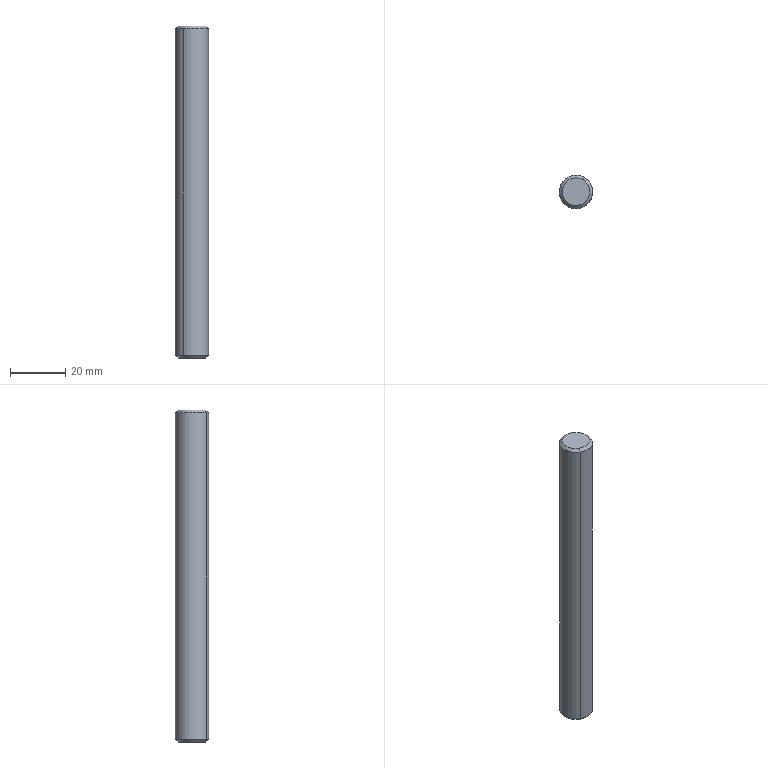Component | SolidWorks | DoubleFilmTransport-1_AdjustmentRod-1 | 1 solid | 8 faces | box 12 x 12 x 120 mm | volume 13536 mm3 | cone 4 | cylinder 2 | plane 2 | commonest cylinder face diameters 12 x2
build123d program:
from build123d import *


with BuildPart() as part:
    # Sketch1 → Revolve1 (revolve)
    with BuildSketch(Plane(origin=(0, 0, 0), x_dir=(1, 0, 0), z_dir=(0, 1, 0))):
        Polygon((5, 60), (0, 60), (0, -60), (5, -60), (6, -59), (6, 59), align=None)
    revolve(axis=Axis((0, 0, -60), (0, 0, 1)))


solid = part.part

# Placed as in the assembly
solid = solid.moved(Location((-298.746, 95.373, -1.5), (0, 0, 0)))
STEP:
#1=COLOUR_RGB('',0.7922,0.8196,0.9333);
#2=FILL_AREA_STYLE_COLOUR('',#1);
#3=FILL_AREA_STYLE('',(#2));
#4=SURFACE_STYLE_FILL_AREA(#3);
#5=SURFACE_SIDE_STYLE('',(#4));
#6=SURFACE_STYLE_USAGE(.BOTH.,#5);
#7=PRESENTATION_STYLE_ASSIGNMENT((#6));
#8=CARTESIAN_POINT('',(-11.863,3.586,2.303));
#9=VERTEX_POINT('',#8);
#10=CARTESIAN_POINT('',(-11.661,3.924,2.303));
#11=VERTEX_POINT('',#10);
#12=CARTESIAN_POINT('',(-11.762,3.755,2.303));
#13=DIRECTION('',(0.,0.,1.));
#14=DIRECTION('',(-0.5123,-0.8588,0.));
#15=AXIS2_PLACEMENT_3D('',#12,#13,#14);
#16=CIRCLE('',#15,0.1969);
#17=EDGE_CURVE('',#9,#11,#16,.T.);
#18=ORIENTED_EDGE('',*,*,#17,.F.);
#19=CARTESIAN_POINT('',(-11.883,3.552,2.264));
#20=VERTEX_POINT('',#19);
#21=CARTESIAN_POINT('',(-11.863,3.586,2.303));
#22=DIRECTION('',(-0.3623,-0.6073,-0.7071));
#23=VECTOR('',#22,39.37);
#24=LINE('',#21,#23);
#25=EDGE_CURVE('',#9,#20,#24,.T.);
#26=ORIENTED_EDGE('',*,*,#25,.T.);
#27=CARTESIAN_POINT('',(-11.641,3.958,2.264));
#28=VERTEX_POINT('',#27);
#29=CARTESIAN_POINT('',(-11.762,3.755,2.264));
#30=DIRECTION('',(0.,0.,1.));
#31=DIRECTION('',(-0.5123,-0.8588,0.));
#32=AXIS2_PLACEMENT_3D('',#29,#30,#31);
#33=CIRCLE('',#32,0.2362);
#34=EDGE_CURVE('',#20,#28,#33,.T.);
#35=ORIENTED_EDGE('',*,*,#34,.T.);
#36=CARTESIAN_POINT('',(-11.661,3.924,2.303));
#37=DIRECTION('',(0.3623,0.6073,-0.7071));
#38=VECTOR('',#37,39.37);
#39=LINE('',#36,#38);
#40=EDGE_CURVE('',#11,#28,#39,.T.);
#41=ORIENTED_EDGE('',*,*,#40,.F.);
#42=EDGE_LOOP('',(#18,#26,#35,#41));
#43=FACE_OUTER_BOUND('',#42,.T.);
#44=CARTESIAN_POINT('',(-11.762,3.755,2.303));
#45=DIRECTION('',(0.,0.,-1.));
#46=DIRECTION('',(0.5123,0.8588,0.));
#47=AXIS2_PLACEMENT_3D('',#44,#45,#46);
#48=CONICAL_SURFACE('',#47,0.1969,0.7854);
#49=ADVANCED_FACE('',(#43),#48,.T.);
#50=CARTESIAN_POINT('',(-11.883,3.552,-2.382));
#51=VERTEX_POINT('',#50);
#52=CARTESIAN_POINT('',(-11.641,3.958,-2.382));
#53=VERTEX_POINT('',#52);
#54=CARTESIAN_POINT('',(-11.762,3.755,-2.382));
#55=DIRECTION('',(0.,0.,1.));
#56=DIRECTION('',(-0.5123,-0.8588,0.));
#57=AXIS2_PLACEMENT_3D('',#54,#55,#56);
#58=CIRCLE('',#57,0.2362);
#59=EDGE_CURVE('',#51,#53,#58,.T.);
#60=ORIENTED_EDGE('',*,*,#59,.T.);
#61=CARTESIAN_POINT('',(-11.641,3.958,-2.421));
#62=DIRECTION('',(0.,0.,1.));
#63=VECTOR('',#62,39.37);
#64=LINE('',#61,#63);
#65=EDGE_CURVE('',#53,#28,#64,.T.);
#66=ORIENTED_EDGE('',*,*,#65,.T.);
#67=ORIENTED_EDGE('',*,*,#34,.F.);
#68=CARTESIAN_POINT('',(-11.883,3.552,-2.421));
#69=DIRECTION('',(0.,0.,1.));
#70=VECTOR('',#69,39.37);
#71=LINE('',#68,#70);
#72=EDGE_CURVE('',#51,#20,#71,.T.);
#73=ORIENTED_EDGE('',*,*,#72,.F.);
#74=EDGE_LOOP('',(#60,#66,#67,#73));
#75=FACE_OUTER_BOUND('',#74,.T.);
#76=CARTESIAN_POINT('',(-11.762,3.755,-2.421));
#77=DIRECTION('',(0.,0.,1.));
#78=DIRECTION('',(-0.5123,-0.8588,0.));
#79=AXIS2_PLACEMENT_3D('',#76,#77,#78);
#80=CYLINDRICAL_SURFACE('',#79,0.2362);
#81=ADVANCED_FACE('',(#75),#80,.T.);
#82=CARTESIAN_POINT('',(-11.863,3.586,-2.421));
#83=VERTEX_POINT('',#82);
#84=CARTESIAN_POINT('',(-11.661,3.924,-2.421));
#85=VERTEX_POINT('',#84);
#86=CARTESIAN_POINT('',(-11.762,3.755,-2.421));
#87=DIRECTION('',(0.,0.,1.));
#88=DIRECTION('',(-0.5123,-0.8588,0.));
#89=AXIS2_PLACEMENT_3D('',#86,#87,#88);
#90=CIRCLE('',#89,0.1969);
#91=EDGE_CURVE('',#83,#85,#90,.T.);
#92=ORIENTED_EDGE('',*,*,#91,.T.);
#93=CARTESIAN_POINT('',(-11.641,3.958,-2.382));
#94=DIRECTION('',(0.3623,0.6073,0.7071));
#95=VECTOR('',#94,39.37);
#96=LINE('',#93,#95);
#97=EDGE_CURVE('',#85,#53,#96,.T.);
#98=ORIENTED_EDGE('',*,*,#97,.T.);
#99=ORIENTED_EDGE('',*,*,#59,.F.);
#100=CARTESIAN_POINT('',(-11.883,3.552,-2.382));
#101=DIRECTION('',(-0.3623,-0.6073,0.7071));
#102=VECTOR('',#101,39.37);
#103=LINE('',#100,#102);
#104=EDGE_CURVE('',#83,#51,#103,.T.);
#105=ORIENTED_EDGE('',*,*,#104,.F.);
#106=EDGE_LOOP('',(#92,#98,#99,#105));
#107=FACE_OUTER_BOUND('',#106,.T.);
#108=CARTESIAN_POINT('',(-11.762,3.755,-2.382));
#109=DIRECTION('',(0.,0.,1.));
#110=DIRECTION('',(-0.5123,-0.8588,0.));
#111=AXIS2_PLACEMENT_3D('',#108,#109,#110);
#112=CONICAL_SURFACE('',#111,0.2362,0.7854);
#113=ADVANCED_FACE('',(#107),#112,.T.);
#114=ORIENTED_EDGE('',*,*,#97,.F.);
#115=CARTESIAN_POINT('',(-11.762,3.755,-2.421));
#116=DIRECTION('',(0.,0.,1.));
#117=DIRECTION('',(-0.5123,-0.8588,0.));
#118=AXIS2_PLACEMENT_3D('',#115,#116,#117);
#119=CIRCLE('',#118,0.1969);
#120=EDGE_CURVE('',#85,#83,#119,.T.);
#121=ORIENTED_EDGE('',*,*,#120,.T.);
#122=ORIENTED_EDGE('',*,*,#104,.T.);
#123=CARTESIAN_POINT('',(-11.762,3.755,-2.382));
#124=DIRECTION('',(0.,0.,1.));
#125=DIRECTION('',(-0.5123,-0.8588,0.));
#126=AXIS2_PLACEMENT_3D('',#123,#124,#125);
#127=CIRCLE('',#126,0.2362);
#128=EDGE_CURVE('',#53,#51,#127,.T.);
#129=ORIENTED_EDGE('',*,*,#128,.F.);
#130=EDGE_LOOP('',(#114,#121,#122,#129));
#131=FACE_OUTER_BOUND('',#130,.T.);
#132=CARTESIAN_POINT('',(-11.762,3.755,-2.382));
#133=DIRECTION('',(0.,0.,1.));
#134=DIRECTION('',(-0.5123,-0.8588,0.));
#135=AXIS2_PLACEMENT_3D('',#132,#133,#134);
#136=CONICAL_SURFACE('',#135,0.2362,0.7854);
#137=ADVANCED_FACE('',(#131),#136,.T.);
#138=ORIENTED_EDGE('',*,*,#65,.F.);
#139=ORIENTED_EDGE('',*,*,#128,.T.);
#140=ORIENTED_EDGE('',*,*,#72,.T.);
#141=CARTESIAN_POINT('',(-11.762,3.755,2.264));
#142=DIRECTION('',(0.,0.,1.));
#143=DIRECTION('',(-0.5123,-0.8588,0.));
#144=AXIS2_PLACEMENT_3D('',#141,#142,#143);
#145=CIRCLE('',#144,0.2362);
#146=EDGE_CURVE('',#28,#20,#145,.T.);
#147=ORIENTED_EDGE('',*,*,#146,.F.);
#148=EDGE_LOOP('',(#138,#139,#140,#147));
#149=FACE_OUTER_BOUND('',#148,.T.);
#150=CARTESIAN_POINT('',(-11.762,3.755,-2.421));
#151=DIRECTION('',(0.,0.,1.));
#152=DIRECTION('',(-0.5123,-0.8588,0.));
#153=AXIS2_PLACEMENT_3D('',#150,#151,#152);
#154=CYLINDRICAL_SURFACE('',#153,0.2362);
#155=ADVANCED_FACE('',(#149),#154,.T.);
#156=ORIENTED_EDGE('',*,*,#25,.F.);
#157=CARTESIAN_POINT('',(-11.762,3.755,2.303));
#158=DIRECTION('',(0.,0.,1.));
#159=DIRECTION('',(-0.5123,-0.8588,0.));
#160=AXIS2_PLACEMENT_3D('',#157,#158,#159);
#161=CIRCLE('',#160,0.1969);
#162=EDGE_CURVE('',#11,#9,#161,.T.);
#163=ORIENTED_EDGE('',*,*,#162,.F.);
#164=ORIENTED_EDGE('',*,*,#40,.T.);
#165=ORIENTED_EDGE('',*,*,#146,.T.);
#166=EDGE_LOOP('',(#156,#163,#164,#165));
#167=FACE_OUTER_BOUND('',#166,.T.);
#168=CARTESIAN_POINT('',(-11.762,3.755,2.303));
#169=DIRECTION('',(0.,0.,-1.));
#170=DIRECTION('',(0.5123,0.8588,0.));
#171=AXIS2_PLACEMENT_3D('',#168,#169,#170);
#172=CONICAL_SURFACE('',#171,0.1969,0.7854);
#173=ADVANCED_FACE('',(#167),#172,.T.);
#174=ORIENTED_EDGE('',*,*,#162,.T.);
#175=ORIENTED_EDGE('',*,*,#17,.T.);
#176=EDGE_LOOP('',(#174,#175));
#177=FACE_OUTER_BOUND('',#176,.T.);
#178=CARTESIAN_POINT('',(-11.762,3.755,2.303));
#179=DIRECTION('',(0.,0.,1.));
#180=DIRECTION('',(-0.5123,-0.8588,0.));
#181=AXIS2_PLACEMENT_3D('',#178,#179,#180);
#182=PLANE('',#181);
#183=ADVANCED_FACE('',(#177),#182,.T.);
#184=ORIENTED_EDGE('',*,*,#91,.F.);
#185=ORIENTED_EDGE('',*,*,#120,.F.);
#186=EDGE_LOOP('',(#184,#185));
#187=FACE_OUTER_BOUND('',#186,.T.);
#188=CARTESIAN_POINT('',(-11.863,3.586,-2.421));
#189=DIRECTION('',(0.,0.,-1.));
#190=DIRECTION('',(0.5123,0.8588,0.));
#191=AXIS2_PLACEMENT_3D('',#188,#189,#190);
#192=PLANE('',#191);
#193=ADVANCED_FACE('',(#187),#192,.T.);
#194=CLOSED_SHELL('',(#49,#81,#113,#137,#155,#173,#183,#193));
#195=MANIFOLD_SOLID_BREP('',#194);
#196=STYLED_ITEM('',(#7),#195);
#197=(LENGTH_UNIT()NAMED_UNIT(*)SI_UNIT($,.METRE.));
#198=LENGTH_MEASURE_WITH_UNIT(LENGTH_MEASURE(0.0254),#197);
#199=DIMENSIONAL_EXPONENTS(1.,0.,0.,0.,0.,0.,0.);
#200=(CONVERSION_BASED_UNIT('',#198)LENGTH_UNIT()NAMED_UNIT(#199));
#201=UNCERTAINTY_MEASURE_WITH_UNIT(LENGTH_MEASURE(0.00001),#200,'','');
#202=(NAMED_UNIT(*)PLANE_ANGLE_UNIT()SI_UNIT($,.RADIAN.));
#203=(NAMED_UNIT(*)SI_UNIT($,.STERADIAN.)SOLID_ANGLE_UNIT());
#204=(GEOMETRIC_REPRESENTATION_CONTEXT(3)GLOBAL_UNCERTAINTY_ASSIGNED_CONTEXT((#201))GLOBAL_UNIT_ASSIGNED_CONTEXT((#200,#202,#203))REPRESENTATION_CONTEXT('',''));
#205=MECHANICAL_DESIGN_GEOMETRIC_PRESENTATION_REPRESENTATION('',(#196),#204);
#206=PRESENTATION_LAYER_ASSIGNMENT('','',(#196));
#207=CARTESIAN_POINT('',(0.,0.,0.));
#208=DIRECTION('',(0.,0.,1.));
#209=DIRECTION('',(1.,0.,0.));
#210=AXIS2_PLACEMENT_3D('',#207,#208,#209);
#211=(LENGTH_UNIT()NAMED_UNIT(*)SI_UNIT($,.METRE.));
#212=LENGTH_MEASURE_WITH_UNIT(LENGTH_MEASURE(0.0254),#211);
#213=DIMENSIONAL_EXPONENTS(1.,0.,0.,0.,0.,0.,0.);
#214=(CONVERSION_BASED_UNIT('',#212)LENGTH_UNIT()NAMED_UNIT(#213));
#215=UNCERTAINTY_MEASURE_WITH_UNIT(LENGTH_MEASURE(0.00001),#214,'','');
#216=(NAMED_UNIT(*)PLANE_ANGLE_UNIT()SI_UNIT($,.RADIAN.));
#217=(NAMED_UNIT(*)SI_UNIT($,.STERADIAN.)SOLID_ANGLE_UNIT());
#218=(GEOMETRIC_REPRESENTATION_CONTEXT(3)GLOBAL_UNCERTAINTY_ASSIGNED_CONTEXT((#215))GLOBAL_UNIT_ASSIGNED_CONTEXT((#214,#216,#217))REPRESENTATION_CONTEXT('',''));
#219=ADVANCED_BREP_SHAPE_REPRESENTATION('',(#195,#210),#218);